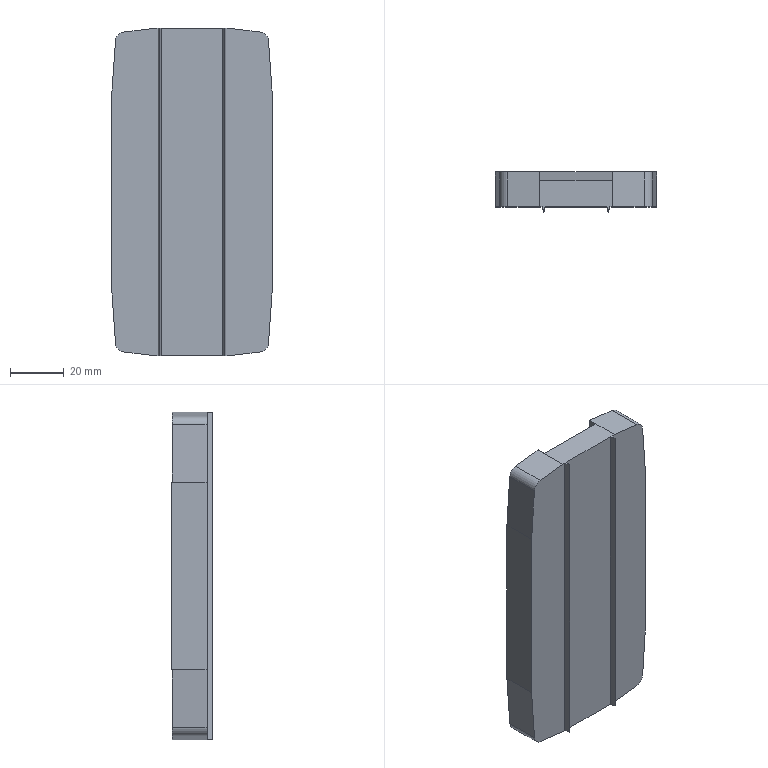Component | SolidWorks | LEFB32T-1800(0_0_0)-1_LEFB32T-1800(0_0_0)2-1 | 1 solid | 74 faces | volume 90341 mm3 | plane 42 | cone 16 | cylinder 16 | commonest cylinder face diameters 4.917 x8 5 x4 7 x4